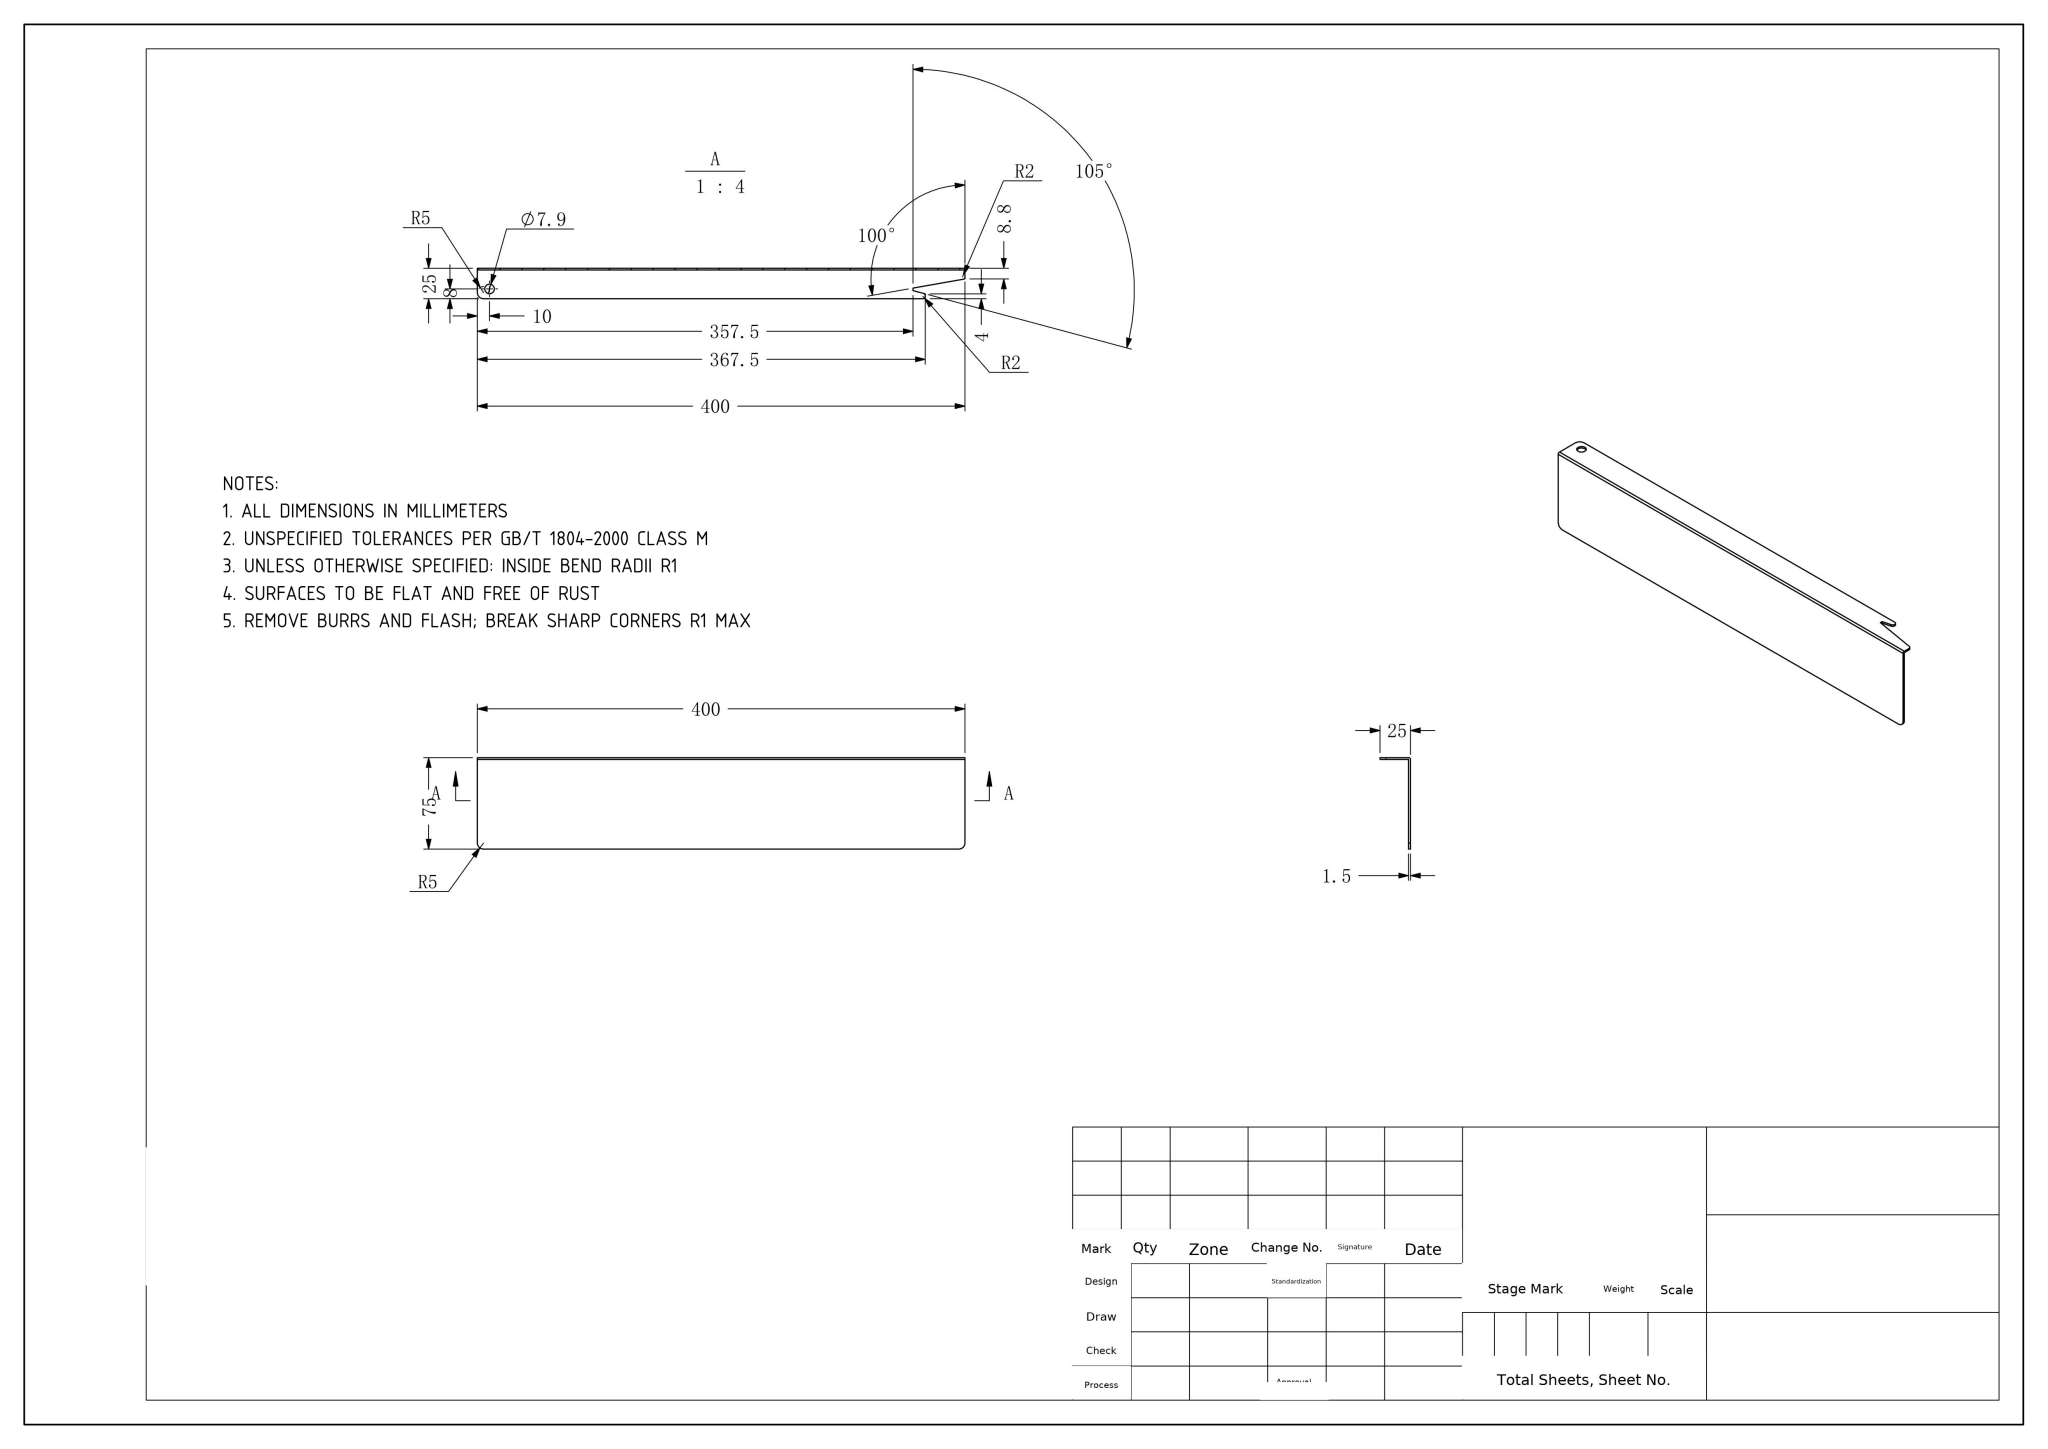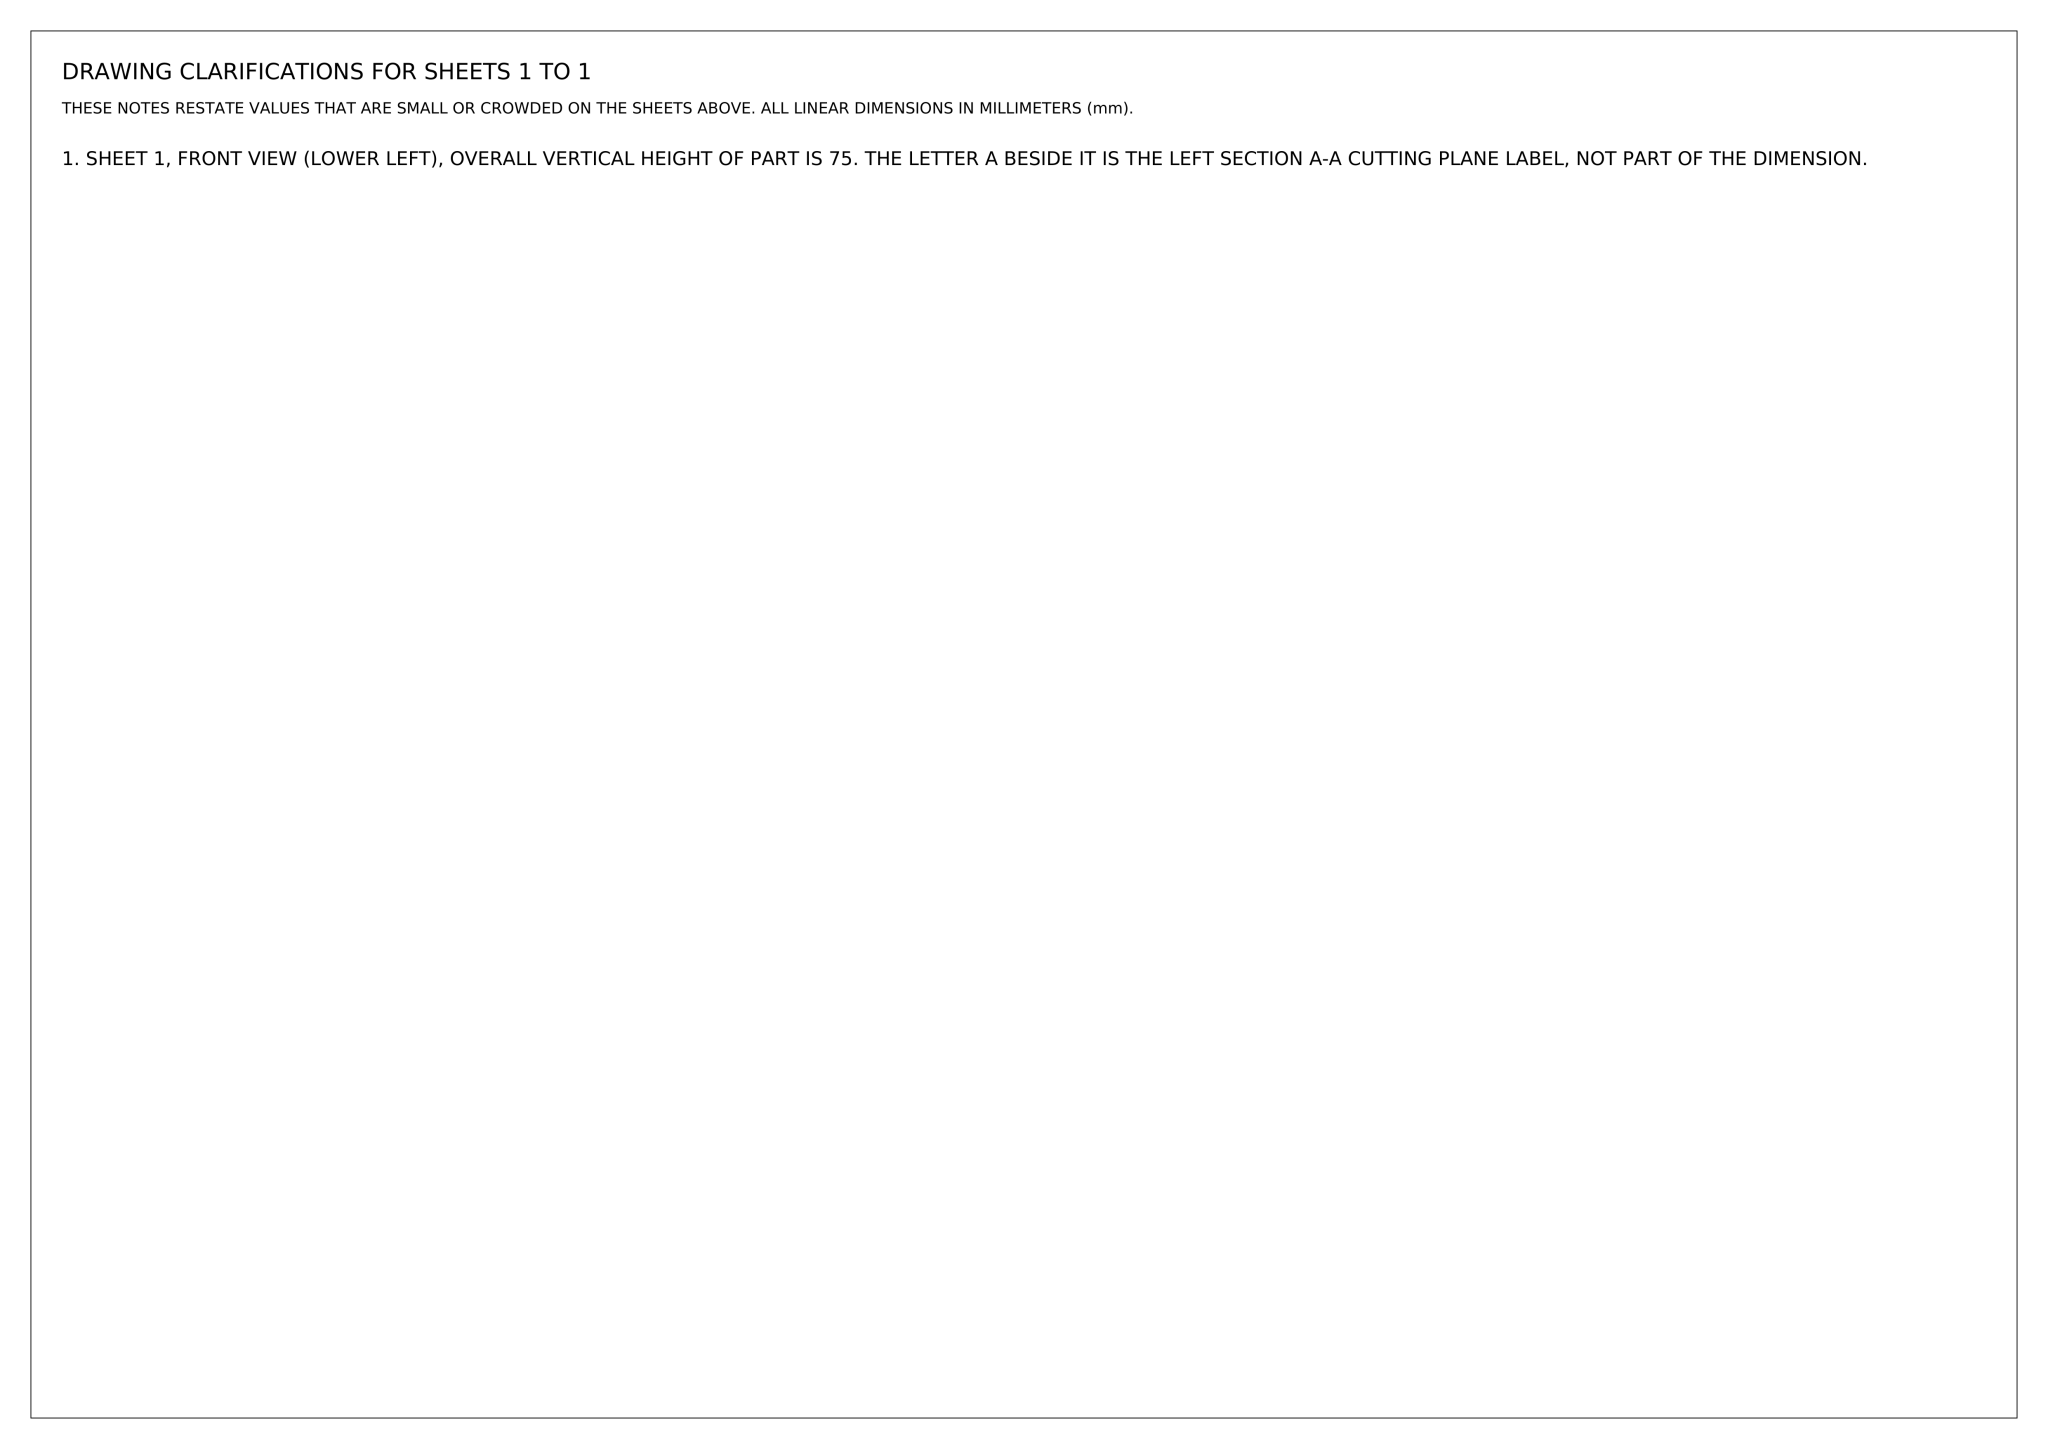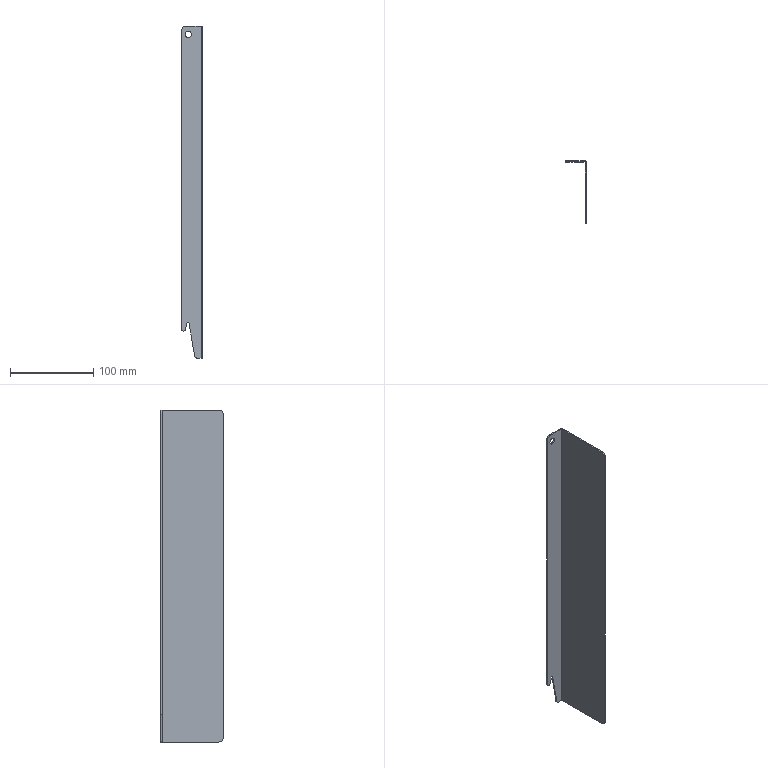Part | NX | mm | Angled Metal Baffle Bracket | 1 solid | 22 faces | box 25 x 75 x 400 mm | volume 58093 mm3 | plane 12 | cylinder 10 | commonest cylinder face diameters 10 x3 4 x3 7.9 x2 3.004 x1 0.004 x1
STEP:
#1=COLOUR_RGB('',0.7529,0.7529,0.7529);
#2=FILL_AREA_STYLE_COLOUR('',#1);
#3=FILL_AREA_STYLE('',(#2));
#4=SURFACE_STYLE_FILL_AREA(#3);
#5=SURFACE_SIDE_STYLE('',(#4));
#6=SURFACE_STYLE_USAGE(.BOTH.,#5);
#7=PRESENTATION_STYLE_ASSIGNMENT((#6));
#8=CARTESIAN_POINT('',(-33.5,-17.5,-31.95));
#9=VERTEX_POINT('',#8);
#10=CARTESIAN_POINT('',(-33.5,-17.5,-24.05));
#11=VERTEX_POINT('',#10);
#12=CARTESIAN_POINT('',(-33.5,-17.5,-28.));
#13=DIRECTION('',(0.,1.,0.));
#14=DIRECTION('',(0.,0.,-1.));
#15=AXIS2_PLACEMENT_3D('',#12,#13,#14);
#16=CIRCLE('',#15,3.95);
#17=EDGE_CURVE('',#9,#11,#16,.T.);
#18=ORIENTED_EDGE('',*,*,#17,.T.);
#19=CARTESIAN_POINT('',(-33.5,-19.,-24.05));
#20=VERTEX_POINT('',#19);
#21=CARTESIAN_POINT('',(-33.5,-17.5,-24.05));
#22=DIRECTION('',(0.,-1.,0.));
#23=VECTOR('',#22,1000.);
#24=LINE('',#21,#23);
#25=EDGE_CURVE('',#11,#20,#24,.T.);
#26=ORIENTED_EDGE('',*,*,#25,.T.);
#27=CARTESIAN_POINT('',(-33.5,-19.,-31.95));
#28=VERTEX_POINT('',#27);
#29=CARTESIAN_POINT('',(-33.5,-19.,-28.));
#30=DIRECTION('',(0.,1.,0.));
#31=DIRECTION('',(0.,0.,-1.));
#32=AXIS2_PLACEMENT_3D('',#29,#30,#31);
#33=CIRCLE('',#32,3.95);
#34=EDGE_CURVE('',#28,#20,#33,.T.);
#35=ORIENTED_EDGE('',*,*,#34,.F.);
#36=CARTESIAN_POINT('',(-33.5,-17.5,-31.95));
#37=DIRECTION('',(0.,-1.,0.));
#38=VECTOR('',#37,1000.);
#39=LINE('',#36,#38);
#40=EDGE_CURVE('',#9,#28,#39,.T.);
#41=ORIENTED_EDGE('',*,*,#40,.F.);
#42=EDGE_LOOP('',(#18,#26,#35,#41));
#43=FACE_OUTER_BOUND('',#42,.T.);
#44=CARTESIAN_POINT('',(-33.5,-17.5,-28.));
#45=DIRECTION('',(0.,-1.,0.));
#46=DIRECTION('',(0.,0.,-1.));
#47=AXIS2_PLACEMENT_3D('',#44,#45,#46);
#48=CYLINDRICAL_SURFACE('',#47,3.95);
#49=ADVANCED_FACE('',(#43),#48,.F.);
#50=CARTESIAN_POINT('',(-18.002,-17.5,-18.));
#51=VERTEX_POINT('',#50);
#52=CARTESIAN_POINT('',(-36.5,-17.5,-18.));
#53=VERTEX_POINT('',#52);
#54=CARTESIAN_POINT('',(-16.5,-17.5,-18.));
#55=DIRECTION('',(-1.,0.,0.));
#56=VECTOR('',#55,1000.);
#57=LINE('',#54,#56);
#58=EDGE_CURVE('',#51,#53,#57,.T.);
#59=ORIENTED_EDGE('',*,*,#58,.T.);
#60=CARTESIAN_POINT('',(-36.5,-19.,-18.));
#61=VERTEX_POINT('',#60);
#62=CARTESIAN_POINT('',(-36.5,-17.5,-18.));
#63=DIRECTION('',(0.,-1.,0.));
#64=VECTOR('',#63,1000.);
#65=LINE('',#62,#64);
#66=EDGE_CURVE('',#53,#61,#65,.T.);
#67=ORIENTED_EDGE('',*,*,#66,.T.);
#68=CARTESIAN_POINT('',(-18.002,-19.,-18.));
#69=VERTEX_POINT('',#68);
#70=CARTESIAN_POINT('',(-16.5,-19.,-18.));
#71=DIRECTION('',(-1.,0.,0.));
#72=VECTOR('',#71,1000.);
#73=LINE('',#70,#72);
#74=EDGE_CURVE('',#69,#61,#73,.T.);
#75=ORIENTED_EDGE('',*,*,#74,.F.);
#76=CARTESIAN_POINT('',(-18.,-19.002,-18.));
#77=VERTEX_POINT('',#76);
#78=CARTESIAN_POINT('',(-18.002,-19.002,-18.));
#79=DIRECTION('',(0.,0.,1.));
#80=DIRECTION('',(-1.,0.,0.));
#81=AXIS2_PLACEMENT_3D('',#78,#79,#80);
#82=CIRCLE('',#81,0.002);
#83=EDGE_CURVE('',#77,#69,#82,.T.);
#84=ORIENTED_EDGE('',*,*,#83,.F.);
#85=CARTESIAN_POINT('',(-18.,-87.5,-18.));
#86=VERTEX_POINT('',#85);
#87=CARTESIAN_POINT('',(-18.,-17.5,-18.));
#88=DIRECTION('',(-0.,1.,0.));
#89=VECTOR('',#88,1000.);
#90=LINE('',#87,#89);
#91=EDGE_CURVE('',#86,#77,#90,.T.);
#92=ORIENTED_EDGE('',*,*,#91,.F.);
#93=CARTESIAN_POINT('',(-16.5,-87.5,-18.));
#94=VERTEX_POINT('',#93);
#95=CARTESIAN_POINT('',(-16.5,-87.5,-18.));
#96=DIRECTION('',(1.,0.,0.));
#97=VECTOR('',#96,1000.);
#98=LINE('',#95,#97);
#99=EDGE_CURVE('',#86,#94,#98,.T.);
#100=ORIENTED_EDGE('',*,*,#99,.T.);
#101=CARTESIAN_POINT('',(-16.5,-19.002,-18.));
#102=VERTEX_POINT('',#101);
#103=CARTESIAN_POINT('',(-16.5,-17.5,-18.));
#104=DIRECTION('',(-0.,1.,0.));
#105=VECTOR('',#104,1000.);
#106=LINE('',#103,#105);
#107=EDGE_CURVE('',#94,#102,#106,.T.);
#108=ORIENTED_EDGE('',*,*,#107,.T.);
#109=CARTESIAN_POINT('',(-18.002,-19.002,-18.));
#110=DIRECTION('',(0.,0.,1.));
#111=DIRECTION('',(-1.,0.,0.));
#112=AXIS2_PLACEMENT_3D('',#109,#110,#111);
#113=CIRCLE('',#112,1.502);
#114=EDGE_CURVE('',#102,#51,#113,.T.);
#115=ORIENTED_EDGE('',*,*,#114,.T.);
#116=EDGE_LOOP('',(#59,#67,#75,#84,#92,#100,#108,#115));
#117=FACE_OUTER_BOUND('',#116,.T.);
#118=CARTESIAN_POINT('',(-16.5,-17.5,-18.));
#119=DIRECTION('',(0.,0.,1.));
#120=DIRECTION('',(-0.,1.,0.));
#121=AXIS2_PLACEMENT_3D('',#118,#119,#120);
#122=PLANE('',#121);
#123=ADVANCED_FACE('',(#117),#122,.T.);
#124=CARTESIAN_POINT('',(-18.,-92.5,-23.));
#125=VERTEX_POINT('',#124);
#126=CARTESIAN_POINT('',(-18.,-92.5,-413.));
#127=VERTEX_POINT('',#126);
#128=CARTESIAN_POINT('',(-18.,-92.5,-18.));
#129=DIRECTION('',(0.,0.,-1.));
#130=VECTOR('',#129,1000.);
#131=LINE('',#128,#130);
#132=EDGE_CURVE('',#125,#127,#131,.T.);
#133=ORIENTED_EDGE('',*,*,#132,.T.);
#134=CARTESIAN_POINT('',(-16.5,-92.5,-413.));
#135=VERTEX_POINT('',#134);
#136=CARTESIAN_POINT('',(-16.5,-92.5,-413.));
#137=DIRECTION('',(1.,0.,0.));
#138=VECTOR('',#137,1000.);
#139=LINE('',#136,#138);
#140=EDGE_CURVE('',#127,#135,#139,.T.);
#141=ORIENTED_EDGE('',*,*,#140,.T.);
#142=CARTESIAN_POINT('',(-16.5,-92.5,-23.));
#143=VERTEX_POINT('',#142);
#144=CARTESIAN_POINT('',(-16.5,-92.5,-18.));
#145=DIRECTION('',(0.,0.,-1.));
#146=VECTOR('',#145,1000.);
#147=LINE('',#144,#146);
#148=EDGE_CURVE('',#143,#135,#147,.T.);
#149=ORIENTED_EDGE('',*,*,#148,.F.);
#150=CARTESIAN_POINT('',(-16.5,-92.5,-23.));
#151=DIRECTION('',(-1.,-0.,0.));
#152=VECTOR('',#151,1000.);
#153=LINE('',#150,#152);
#154=EDGE_CURVE('',#143,#125,#153,.T.);
#155=ORIENTED_EDGE('',*,*,#154,.T.);
#156=EDGE_LOOP('',(#133,#141,#149,#155));
#157=FACE_OUTER_BOUND('',#156,.T.);
#158=CARTESIAN_POINT('',(-16.5,-92.5,-18.));
#159=DIRECTION('',(-0.,1.,0.));
#160=DIRECTION('',(0.,0.,-1.));
#161=AXIS2_PLACEMENT_3D('',#158,#159,#160);
#162=PLANE('',#161);
#163=ADVANCED_FACE('',(#157),#162,.F.);
#164=CARTESIAN_POINT('',(-18.002,-19.,-418.));
#165=VERTEX_POINT('',#164);
#166=CARTESIAN_POINT('',(-23.645,-19.,-418.));
#167=VERTEX_POINT('',#166);
#168=CARTESIAN_POINT('',(-16.5,-19.,-418.));
#169=DIRECTION('',(-1.,0.,0.));
#170=VECTOR('',#169,1000.);
#171=LINE('',#168,#170);
#172=EDGE_CURVE('',#165,#167,#171,.T.);
#173=ORIENTED_EDGE('',*,*,#172,.T.);
#174=CARTESIAN_POINT('',(-23.645,-17.5,-418.));
#175=VERTEX_POINT('',#174);
#176=CARTESIAN_POINT('',(-23.645,-17.5,-418.));
#177=DIRECTION('',(0.,1.,0.));
#178=VECTOR('',#177,1000.);
#179=LINE('',#176,#178);
#180=EDGE_CURVE('',#167,#175,#179,.T.);
#181=ORIENTED_EDGE('',*,*,#180,.T.);
#182=CARTESIAN_POINT('',(-18.002,-17.5,-418.));
#183=VERTEX_POINT('',#182);
#184=CARTESIAN_POINT('',(-16.5,-17.5,-418.));
#185=DIRECTION('',(-1.,0.,0.));
#186=VECTOR('',#185,1000.);
#187=LINE('',#184,#186);
#188=EDGE_CURVE('',#183,#175,#187,.T.);
#189=ORIENTED_EDGE('',*,*,#188,.F.);
#190=CARTESIAN_POINT('',(-16.5,-19.002,-418.));
#191=VERTEX_POINT('',#190);
#192=CARTESIAN_POINT('',(-18.002,-19.002,-418.));
#193=DIRECTION('',(0.,0.,1.));
#194=DIRECTION('',(-1.,0.,0.));
#195=AXIS2_PLACEMENT_3D('',#192,#193,#194);
#196=CIRCLE('',#195,1.502);
#197=EDGE_CURVE('',#191,#183,#196,.T.);
#198=ORIENTED_EDGE('',*,*,#197,.F.);
#199=CARTESIAN_POINT('',(-16.5,-87.5,-418.));
#200=VERTEX_POINT('',#199);
#201=CARTESIAN_POINT('',(-16.5,-17.5,-418.));
#202=DIRECTION('',(-0.,1.,0.));
#203=VECTOR('',#202,1000.);
#204=LINE('',#201,#203);
#205=EDGE_CURVE('',#200,#191,#204,.T.);
#206=ORIENTED_EDGE('',*,*,#205,.F.);
#207=CARTESIAN_POINT('',(-18.,-87.5,-418.));
#208=VERTEX_POINT('',#207);
#209=CARTESIAN_POINT('',(-16.5,-87.5,-418.));
#210=DIRECTION('',(-1.,-0.,0.));
#211=VECTOR('',#210,1000.);
#212=LINE('',#209,#211);
#213=EDGE_CURVE('',#200,#208,#212,.T.);
#214=ORIENTED_EDGE('',*,*,#213,.T.);
#215=CARTESIAN_POINT('',(-18.,-19.002,-418.));
#216=VERTEX_POINT('',#215);
#217=CARTESIAN_POINT('',(-18.,-17.5,-418.));
#218=DIRECTION('',(-0.,1.,0.));
#219=VECTOR('',#218,1000.);
#220=LINE('',#217,#219);
#221=EDGE_CURVE('',#208,#216,#220,.T.);
#222=ORIENTED_EDGE('',*,*,#221,.T.);
#223=CARTESIAN_POINT('',(-18.002,-19.002,-418.));
#224=DIRECTION('',(0.,0.,1.));
#225=DIRECTION('',(-1.,0.,0.));
#226=AXIS2_PLACEMENT_3D('',#223,#224,#225);
#227=CIRCLE('',#226,0.002);
#228=EDGE_CURVE('',#216,#165,#227,.T.);
#229=ORIENTED_EDGE('',*,*,#228,.T.);
#230=EDGE_LOOP('',(#173,#181,#189,#198,#206,#214,#222,#229));
#231=FACE_OUTER_BOUND('',#230,.T.);
#232=CARTESIAN_POINT('',(-16.5,-17.5,-418.));
#233=DIRECTION('',(0.,0.,1.));
#234=DIRECTION('',(-1.,0.,0.));
#235=AXIS2_PLACEMENT_3D('',#232,#233,#234);
#236=PLANE('',#235);
#237=ADVANCED_FACE('',(#231),#236,.F.);
#238=ORIENTED_EDGE('',*,*,#17,.F.);
#239=CARTESIAN_POINT('',(-33.5,-17.5,-28.));
#240=DIRECTION('',(0.,1.,0.));
#241=DIRECTION('',(0.,0.,-1.));
#242=AXIS2_PLACEMENT_3D('',#239,#240,#241);
#243=CIRCLE('',#242,3.95);
#244=EDGE_CURVE('',#11,#9,#243,.T.);
#245=ORIENTED_EDGE('',*,*,#244,.F.);
#246=EDGE_LOOP('',(#238,#245));
#247=FACE_BOUND('',#246,.T.);
#248=CARTESIAN_POINT('',(-39.5,-17.5,-385.479));
#249=VERTEX_POINT('',#248);
#250=CARTESIAN_POINT('',(-39.035,-17.5,-385.479));
#251=VERTEX_POINT('',#250);
#252=CARTESIAN_POINT('',(-16.5,-17.5,-385.479));
#253=DIRECTION('',(1.,0.,0.));
#254=VECTOR('',#253,1000.);
#255=LINE('',#252,#254);
#256=EDGE_CURVE('',#249,#251,#255,.T.);
#257=ORIENTED_EDGE('',*,*,#256,.F.);
#258=CARTESIAN_POINT('',(-41.5,-17.5,-383.479));
#259=VERTEX_POINT('',#258);
#260=CARTESIAN_POINT('',(-39.5,-17.5,-383.479));
#261=DIRECTION('',(0.,1.,0.));
#262=DIRECTION('',(0.,0.,-1.));
#263=AXIS2_PLACEMENT_3D('',#260,#261,#262);
#264=CIRCLE('',#263,2.);
#265=EDGE_CURVE('',#249,#259,#264,.T.);
#266=ORIENTED_EDGE('',*,*,#265,.T.);
#267=CARTESIAN_POINT('',(-41.5,-17.5,-23.));
#268=VERTEX_POINT('',#267);
#269=CARTESIAN_POINT('',(-41.5,-17.5,-18.));
#270=DIRECTION('',(0.,0.,-1.));
#271=VECTOR('',#270,1000.);
#272=LINE('',#269,#271);
#273=EDGE_CURVE('',#268,#259,#272,.T.);
#274=ORIENTED_EDGE('',*,*,#273,.F.);
#275=CARTESIAN_POINT('',(-36.5,-17.5,-23.));
#276=DIRECTION('',(0.,1.,0.));
#277=DIRECTION('',(0.,0.,-1.));
#278=AXIS2_PLACEMENT_3D('',#275,#276,#277);
#279=CIRCLE('',#278,5.);
#280=EDGE_CURVE('',#268,#53,#279,.T.);
#281=ORIENTED_EDGE('',*,*,#280,.T.);
#282=ORIENTED_EDGE('',*,*,#58,.F.);
#283=CARTESIAN_POINT('',(-18.002,-17.5,-18.));
#284=DIRECTION('',(0.,0.,-1.));
#285=VECTOR('',#284,1000.);
#286=LINE('',#283,#285);
#287=EDGE_CURVE('',#51,#183,#286,.T.);
#288=ORIENTED_EDGE('',*,*,#287,.T.);
#289=ORIENTED_EDGE('',*,*,#188,.T.);
#290=CARTESIAN_POINT('',(-25.614,-17.5,-416.347));
#291=VERTEX_POINT('',#290);
#292=CARTESIAN_POINT('',(-23.645,-17.5,-416.));
#293=DIRECTION('',(0.,1.,0.));
#294=DIRECTION('',(0.,0.,-1.));
#295=AXIS2_PLACEMENT_3D('',#292,#293,#294);
#296=CIRCLE('',#295,2.);
#297=EDGE_CURVE('',#175,#291,#296,.T.);
#298=ORIENTED_EDGE('',*,*,#297,.T.);
#299=CARTESIAN_POINT('',(-32.821,-17.5,-375.479));
#300=VERTEX_POINT('',#299);
#301=CARTESIAN_POINT('',(-93.461,-17.5,-31.57));
#302=DIRECTION('',(0.1736,0.,-0.9848));
#303=VECTOR('',#302,1000.);
#304=LINE('',#301,#303);
#305=EDGE_CURVE('',#300,#291,#304,.T.);
#306=ORIENTED_EDGE('',*,*,#305,.F.);
#307=CARTESIAN_POINT('',(-34.821,-17.5,-375.479));
#308=VERTEX_POINT('',#307);
#309=CARTESIAN_POINT('',(-16.5,-17.5,-375.479));
#310=DIRECTION('',(1.,0.,0.));
#311=VECTOR('',#310,1000.);
#312=LINE('',#309,#311);
#313=EDGE_CURVE('',#308,#300,#312,.T.);
#314=ORIENTED_EDGE('',*,*,#313,.F.);
#315=CARTESIAN_POINT('',(-37.103,-17.5,-383.997));
#316=VERTEX_POINT('',#315);
#317=CARTESIAN_POINT('',(55.776,-17.5,-37.366));
#318=DIRECTION('',(0.2588,0.,0.9659));
#319=VECTOR('',#318,1000.);
#320=LINE('',#317,#319);
#321=EDGE_CURVE('',#316,#308,#320,.T.);
#322=ORIENTED_EDGE('',*,*,#321,.F.);
#323=CARTESIAN_POINT('',(-39.035,-17.5,-383.479));
#324=DIRECTION('',(0.,1.,0.));
#325=DIRECTION('',(-0.,0.,-1.));
#326=AXIS2_PLACEMENT_3D('',#323,#324,#325);
#327=CIRCLE('',#326,2.);
#328=EDGE_CURVE('',#316,#251,#327,.T.);
#329=ORIENTED_EDGE('',*,*,#328,.T.);
#330=EDGE_LOOP('',(#257,#266,#274,#281,#282,#288,#289,#298,#306,#314,#322,#329));
#331=FACE_OUTER_BOUND('',#330,.T.);
#332=CARTESIAN_POINT('',(-16.5,-17.5,-18.));
#333=DIRECTION('',(0.,-1.,0.));
#334=DIRECTION('',(0.,0.,-1.));
#335=AXIS2_PLACEMENT_3D('',#332,#333,#334);
#336=PLANE('',#335);
#337=ADVANCED_FACE('',(#247,#331),#336,.F.);
#338=ORIENTED_EDGE('',*,*,#148,.T.);
#339=CARTESIAN_POINT('',(-16.5,-87.5,-413.));
#340=DIRECTION('',(1.,0.,0.));
#341=DIRECTION('',(0.,-1.,0.));
#342=AXIS2_PLACEMENT_3D('',#339,#340,#341);
#343=CIRCLE('',#342,5.);
#344=EDGE_CURVE('',#135,#200,#343,.T.);
#345=ORIENTED_EDGE('',*,*,#344,.T.);
#346=ORIENTED_EDGE('',*,*,#205,.T.);
#347=CARTESIAN_POINT('',(-16.5,-19.002,-18.));
#348=DIRECTION('',(0.,0.,-1.));
#349=VECTOR('',#348,1000.);
#350=LINE('',#347,#349);
#351=EDGE_CURVE('',#102,#191,#350,.T.);
#352=ORIENTED_EDGE('',*,*,#351,.F.);
#353=ORIENTED_EDGE('',*,*,#107,.F.);
#354=CARTESIAN_POINT('',(-16.5,-87.5,-23.));
#355=DIRECTION('',(1.,0.,0.));
#356=DIRECTION('',(0.,-1.,0.));
#357=AXIS2_PLACEMENT_3D('',#354,#355,#356);
#358=CIRCLE('',#357,5.);
#359=EDGE_CURVE('',#94,#143,#358,.T.);
#360=ORIENTED_EDGE('',*,*,#359,.T.);
#361=EDGE_LOOP('',(#338,#345,#346,#352,#353,#360));
#362=FACE_OUTER_BOUND('',#361,.T.);
#363=CARTESIAN_POINT('',(-16.5,-17.5,-18.));
#364=DIRECTION('',(-1.,-0.,0.));
#365=DIRECTION('',(0.,-1.,0.));
#366=AXIS2_PLACEMENT_3D('',#363,#364,#365);
#367=PLANE('',#366);
#368=ADVANCED_FACE('',(#362),#367,.F.);
#369=ORIENTED_EDGE('',*,*,#197,.T.);
#370=ORIENTED_EDGE('',*,*,#287,.F.);
#371=ORIENTED_EDGE('',*,*,#114,.F.);
#372=ORIENTED_EDGE('',*,*,#351,.T.);
#373=EDGE_LOOP('',(#369,#370,#371,#372));
#374=FACE_OUTER_BOUND('',#373,.T.);
#375=CARTESIAN_POINT('',(-18.002,-19.002,-18.));
#376=DIRECTION('',(0.,0.,-1.));
#377=DIRECTION('',(-1.,0.,0.));
#378=AXIS2_PLACEMENT_3D('',#375,#376,#377);
#379=CYLINDRICAL_SURFACE('',#378,1.502);
#380=ADVANCED_FACE('',(#374),#379,.T.);
#381=ORIENTED_EDGE('',*,*,#273,.T.);
#382=CARTESIAN_POINT('',(-41.5,-19.,-383.479));
#383=VERTEX_POINT('',#382);
#384=CARTESIAN_POINT('',(-41.5,-19.,-383.479));
#385=DIRECTION('',(0.,-1.,0.));
#386=VECTOR('',#385,1000.);
#387=LINE('',#384,#386);
#388=EDGE_CURVE('',#259,#383,#387,.T.);
#389=ORIENTED_EDGE('',*,*,#388,.T.);
#390=CARTESIAN_POINT('',(-41.5,-19.,-23.));
#391=VERTEX_POINT('',#390);
#392=CARTESIAN_POINT('',(-41.5,-19.,-18.));
#393=DIRECTION('',(0.,0.,-1.));
#394=VECTOR('',#393,1000.);
#395=LINE('',#392,#394);
#396=EDGE_CURVE('',#391,#383,#395,.T.);
#397=ORIENTED_EDGE('',*,*,#396,.F.);
#398=CARTESIAN_POINT('',(-41.5,-17.5,-23.));
#399=DIRECTION('',(0.,1.,0.));
#400=VECTOR('',#399,1000.);
#401=LINE('',#398,#400);
#402=EDGE_CURVE('',#391,#268,#401,.T.);
#403=ORIENTED_EDGE('',*,*,#402,.T.);
#404=EDGE_LOOP('',(#381,#389,#397,#403));
#405=FACE_OUTER_BOUND('',#404,.T.);
#406=CARTESIAN_POINT('',(-41.5,-17.5,-18.));
#407=DIRECTION('',(-1.,0.,0.));
#408=DIRECTION('',(0.,0.,-1.));
#409=AXIS2_PLACEMENT_3D('',#406,#407,#408);
#410=PLANE('',#409);
#411=ADVANCED_FACE('',(#405),#410,.T.);
#412=ORIENTED_EDGE('',*,*,#396,.T.);
#413=CARTESIAN_POINT('',(-39.5,-19.,-385.479));
#414=VERTEX_POINT('',#413);
#415=CARTESIAN_POINT('',(-39.5,-19.,-383.479));
#416=DIRECTION('',(0.,-1.,0.));
#417=DIRECTION('',(0.,0.,-1.));
#418=AXIS2_PLACEMENT_3D('',#415,#416,#417);
#419=CIRCLE('',#418,2.);
#420=EDGE_CURVE('',#383,#414,#419,.T.);
#421=ORIENTED_EDGE('',*,*,#420,.T.);
#422=CARTESIAN_POINT('',(-39.035,-19.,-385.479));
#423=VERTEX_POINT('',#422);
#424=CARTESIAN_POINT('',(-16.5,-19.,-385.479));
#425=DIRECTION('',(1.,0.,0.));
#426=VECTOR('',#425,1000.);
#427=LINE('',#424,#426);
#428=EDGE_CURVE('',#414,#423,#427,.T.);
#429=ORIENTED_EDGE('',*,*,#428,.T.);
#430=CARTESIAN_POINT('',(-37.103,-19.,-383.997));
#431=VERTEX_POINT('',#430);
#432=CARTESIAN_POINT('',(-39.035,-19.,-383.479));
#433=DIRECTION('',(0.,-1.,0.));
#434=DIRECTION('',(0.,0.,-1.));
#435=AXIS2_PLACEMENT_3D('',#432,#433,#434);
#436=CIRCLE('',#435,2.);
#437=EDGE_CURVE('',#423,#431,#436,.T.);
#438=ORIENTED_EDGE('',*,*,#437,.T.);
#439=CARTESIAN_POINT('',(-34.821,-19.,-375.479));
#440=VERTEX_POINT('',#439);
#441=CARTESIAN_POINT('',(55.776,-19.,-37.366));
#442=DIRECTION('',(0.2588,0.,0.9659));
#443=VECTOR('',#442,1000.);
#444=LINE('',#441,#443);
#445=EDGE_CURVE('',#431,#440,#444,.T.);
#446=ORIENTED_EDGE('',*,*,#445,.T.);
#447=CARTESIAN_POINT('',(-32.821,-19.,-375.479));
#448=VERTEX_POINT('',#447);
#449=CARTESIAN_POINT('',(-16.5,-19.,-375.479));
#450=DIRECTION('',(1.,0.,0.));
#451=VECTOR('',#450,1000.);
#452=LINE('',#449,#451);
#453=EDGE_CURVE('',#440,#448,#452,.T.);
#454=ORIENTED_EDGE('',*,*,#453,.T.);
#455=CARTESIAN_POINT('',(-25.614,-19.,-416.347));
#456=VERTEX_POINT('',#455);
#457=CARTESIAN_POINT('',(-93.461,-19.,-31.57));
#458=DIRECTION('',(0.1736,0.,-0.9848));
#459=VECTOR('',#458,1000.);
#460=LINE('',#457,#459);
#461=EDGE_CURVE('',#448,#456,#460,.T.);
#462=ORIENTED_EDGE('',*,*,#461,.T.);
#463=CARTESIAN_POINT('',(-23.645,-19.,-416.));
#464=DIRECTION('',(0.,-1.,0.));
#465=DIRECTION('',(0.,0.,-1.));
#466=AXIS2_PLACEMENT_3D('',#463,#464,#465);
#467=CIRCLE('',#466,2.);
#468=EDGE_CURVE('',#456,#167,#467,.T.);
#469=ORIENTED_EDGE('',*,*,#468,.T.);
#470=ORIENTED_EDGE('',*,*,#172,.F.);
#471=CARTESIAN_POINT('',(-18.002,-19.,-18.));
#472=DIRECTION('',(0.,0.,-1.));
#473=VECTOR('',#472,1000.);
#474=LINE('',#471,#473);
#475=EDGE_CURVE('',#69,#165,#474,.T.);
#476=ORIENTED_EDGE('',*,*,#475,.F.);
#477=ORIENTED_EDGE('',*,*,#74,.T.);
#478=CARTESIAN_POINT('',(-36.5,-19.,-23.));
#479=DIRECTION('',(0.,-1.,0.));
#480=DIRECTION('',(0.,0.,-1.));
#481=AXIS2_PLACEMENT_3D('',#478,#479,#480);
#482=CIRCLE('',#481,5.);
#483=EDGE_CURVE('',#61,#391,#482,.T.);
#484=ORIENTED_EDGE('',*,*,#483,.T.);
#485=EDGE_LOOP('',(#412,#421,#429,#438,#446,#454,#462,#469,#470,#476,#477,#484));
#486=FACE_OUTER_BOUND('',#485,.T.);
#487=ORIENTED_EDGE('',*,*,#34,.T.);
#488=CARTESIAN_POINT('',(-33.5,-19.,-28.));
#489=DIRECTION('',(0.,1.,0.));
#490=DIRECTION('',(0.,0.,-1.));
#491=AXIS2_PLACEMENT_3D('',#488,#489,#490);
#492=CIRCLE('',#491,3.95);
#493=EDGE_CURVE('',#20,#28,#492,.T.);
#494=ORIENTED_EDGE('',*,*,#493,.T.);
#495=EDGE_LOOP('',(#487,#494));
#496=FACE_BOUND('',#495,.T.);
#497=CARTESIAN_POINT('',(-16.5,-19.,-18.));
#498=DIRECTION('',(0.,-1.,0.));
#499=DIRECTION('',(0.,0.,-1.));
#500=AXIS2_PLACEMENT_3D('',#497,#498,#499);
#501=PLANE('',#500);
#502=ADVANCED_FACE('',(#486,#496),#501,.T.);
#503=ORIENTED_EDGE('',*,*,#221,.F.);
#504=CARTESIAN_POINT('',(-18.,-87.5,-413.));
#505=DIRECTION('',(-1.,-0.,0.));
#506=DIRECTION('',(0.,-1.,0.));
#507=AXIS2_PLACEMENT_3D('',#504,#505,#506);
#508=CIRCLE('',#507,5.);
#509=EDGE_CURVE('',#208,#127,#508,.T.);
#510=ORIENTED_EDGE('',*,*,#509,.T.);
#511=ORIENTED_EDGE('',*,*,#132,.F.);
#512=CARTESIAN_POINT('',(-18.,-87.5,-23.));
#513=DIRECTION('',(-1.,-0.,0.));
#514=DIRECTION('',(0.,-1.,0.));
#515=AXIS2_PLACEMENT_3D('',#512,#513,#514);
#516=CIRCLE('',#515,5.);
#517=EDGE_CURVE('',#125,#86,#516,.T.);
#518=ORIENTED_EDGE('',*,*,#517,.T.);
#519=ORIENTED_EDGE('',*,*,#91,.T.);
#520=CARTESIAN_POINT('',(-18.,-19.002,-18.));
#521=DIRECTION('',(0.,0.,-1.));
#522=VECTOR('',#521,1000.);
#523=LINE('',#520,#522);
#524=EDGE_CURVE('',#77,#216,#523,.T.);
#525=ORIENTED_EDGE('',*,*,#524,.T.);
#526=EDGE_LOOP('',(#503,#510,#511,#518,#519,#525));
#527=FACE_OUTER_BOUND('',#526,.T.);
#528=CARTESIAN_POINT('',(-18.,-17.5,-18.));
#529=DIRECTION('',(-1.,-0.,0.));
#530=DIRECTION('',(0.,-1.,0.));
#531=AXIS2_PLACEMENT_3D('',#528,#529,#530);
#532=PLANE('',#531);
#533=ADVANCED_FACE('',(#527),#532,.T.);
#534=ORIENTED_EDGE('',*,*,#228,.F.);
#535=ORIENTED_EDGE('',*,*,#524,.F.);
#536=ORIENTED_EDGE('',*,*,#83,.T.);
#537=ORIENTED_EDGE('',*,*,#475,.T.);
#538=EDGE_LOOP('',(#534,#535,#536,#537));
#539=FACE_OUTER_BOUND('',#538,.T.);
#540=CARTESIAN_POINT('',(-18.002,-19.002,-18.));
#541=DIRECTION('',(0.,0.,-1.));
#542=DIRECTION('',(-1.,0.,0.));
#543=AXIS2_PLACEMENT_3D('',#540,#541,#542);
#544=CYLINDRICAL_SURFACE('',#543,0.002);
#545=ADVANCED_FACE('',(#539),#544,.F.);
#546=ORIENTED_EDGE('',*,*,#25,.F.);
#547=ORIENTED_EDGE('',*,*,#244,.T.);
#548=ORIENTED_EDGE('',*,*,#40,.T.);
#549=ORIENTED_EDGE('',*,*,#493,.F.);
#550=EDGE_LOOP('',(#546,#547,#548,#549));
#551=FACE_OUTER_BOUND('',#550,.T.);
#552=CARTESIAN_POINT('',(-33.5,-17.5,-28.));
#553=DIRECTION('',(0.,-1.,0.));
#554=DIRECTION('',(0.,0.,-1.));
#555=AXIS2_PLACEMENT_3D('',#552,#553,#554);
#556=CYLINDRICAL_SURFACE('',#555,3.95);
#557=ADVANCED_FACE('',(#551),#556,.F.);
#558=ORIENTED_EDGE('',*,*,#428,.F.);
#559=CARTESIAN_POINT('',(-39.5,-17.5,-385.479));
#560=DIRECTION('',(0.,1.,0.));
#561=VECTOR('',#560,1000.);
#562=LINE('',#559,#561);
#563=EDGE_CURVE('',#414,#249,#562,.T.);
#564=ORIENTED_EDGE('',*,*,#563,.T.);
#565=ORIENTED_EDGE('',*,*,#256,.T.);
#566=CARTESIAN_POINT('',(-39.035,-17.5,-385.479));
#567=DIRECTION('',(0.,-1.,0.));
#568=VECTOR('',#567,1000.);
#569=LINE('',#566,#568);
#570=EDGE_CURVE('',#251,#423,#569,.T.);
#571=ORIENTED_EDGE('',*,*,#570,.T.);
#572=EDGE_LOOP('',(#558,#564,#565,#571));
#573=FACE_OUTER_BOUND('',#572,.T.);
#574=CARTESIAN_POINT('',(-16.5,-17.5,-385.479));
#575=DIRECTION('',(0.,0.,-1.));
#576=DIRECTION('',(1.,0.,0.));
#577=AXIS2_PLACEMENT_3D('',#574,#575,#576);
#578=PLANE('',#577);
#579=ADVANCED_FACE('',(#573),#578,.T.);
#580=ORIENTED_EDGE('',*,*,#445,.F.);
#581=CARTESIAN_POINT('',(-37.103,-17.5,-383.997));
#582=DIRECTION('',(0.,1.,0.));
#583=VECTOR('',#582,1000.);
#584=LINE('',#581,#583);
#585=EDGE_CURVE('',#431,#316,#584,.T.);
#586=ORIENTED_EDGE('',*,*,#585,.T.);
#587=ORIENTED_EDGE('',*,*,#321,.T.);
#588=CARTESIAN_POINT('',(-34.821,-17.5,-375.479));
#589=DIRECTION('',(0.,1.,0.));
#590=VECTOR('',#589,1000.);
#591=LINE('',#588,#590);
#592=EDGE_CURVE('',#440,#308,#591,.T.);
#593=ORIENTED_EDGE('',*,*,#592,.F.);
#594=EDGE_LOOP('',(#580,#586,#587,#593));
#595=FACE_OUTER_BOUND('',#594,.T.);
#596=CARTESIAN_POINT('',(55.776,-17.5,-37.366));
#597=DIRECTION('',(0.9659,0.,-0.2588));
#598=DIRECTION('',(0.2588,0.,0.9659));
#599=AXIS2_PLACEMENT_3D('',#596,#597,#598);
#600=PLANE('',#599);
#601=ADVANCED_FACE('',(#595),#600,.T.);
#602=ORIENTED_EDGE('',*,*,#592,.T.);
#603=ORIENTED_EDGE('',*,*,#313,.T.);
#604=CARTESIAN_POINT('',(-32.821,-17.5,-375.479));
#605=DIRECTION('',(0.,1.,0.));
#606=VECTOR('',#605,1000.);
#607=LINE('',#604,#606);
#608=EDGE_CURVE('',#448,#300,#607,.T.);
#609=ORIENTED_EDGE('',*,*,#608,.F.);
#610=ORIENTED_EDGE('',*,*,#453,.F.);
#611=EDGE_LOOP('',(#602,#603,#609,#610));
#612=FACE_OUTER_BOUND('',#611,.T.);
#613=CARTESIAN_POINT('',(-16.5,-17.5,-375.479));
#614=DIRECTION('',(0.,0.,-1.));
#615=DIRECTION('',(1.,0.,0.));
#616=AXIS2_PLACEMENT_3D('',#613,#614,#615);
#617=PLANE('',#616);
#618=ADVANCED_FACE('',(#612),#617,.T.);
#619=ORIENTED_EDGE('',*,*,#305,.T.);
#620=CARTESIAN_POINT('',(-25.614,-19.,-416.347));
#621=DIRECTION('',(0.,-1.,0.));
#622=VECTOR('',#621,1000.);
#623=LINE('',#620,#622);
#624=EDGE_CURVE('',#291,#456,#623,.T.);
#625=ORIENTED_EDGE('',*,*,#624,.T.);
#626=ORIENTED_EDGE('',*,*,#461,.F.);
#627=ORIENTED_EDGE('',*,*,#608,.T.);
#628=EDGE_LOOP('',(#619,#625,#626,#627));
#629=FACE_OUTER_BOUND('',#628,.T.);
#630=CARTESIAN_POINT('',(-93.461,-17.5,-31.57));
#631=DIRECTION('',(-0.9848,0.,-0.1736));
#632=DIRECTION('',(0.1736,0.,-0.9848));
#633=AXIS2_PLACEMENT_3D('',#630,#631,#632);
#634=PLANE('',#633);
#635=ADVANCED_FACE('',(#629),#634,.T.);
#636=ORIENTED_EDGE('',*,*,#509,.F.);
#637=ORIENTED_EDGE('',*,*,#213,.F.);
#638=ORIENTED_EDGE('',*,*,#344,.F.);
#639=ORIENTED_EDGE('',*,*,#140,.F.);
#640=EDGE_LOOP('',(#636,#637,#638,#639));
#641=FACE_OUTER_BOUND('',#640,.T.);
#642=CARTESIAN_POINT('',(-16.5,-87.5,-413.));
#643=DIRECTION('',(1.,0.,0.));
#644=DIRECTION('',(0.,1.,0.));
#645=AXIS2_PLACEMENT_3D('',#642,#643,#644);
#646=CYLINDRICAL_SURFACE('',#645,5.);
#647=ADVANCED_FACE('',(#641),#646,.T.);
#648=ORIENTED_EDGE('',*,*,#483,.F.);
#649=ORIENTED_EDGE('',*,*,#66,.F.);
#650=ORIENTED_EDGE('',*,*,#280,.F.);
#651=ORIENTED_EDGE('',*,*,#402,.F.);
#652=EDGE_LOOP('',(#648,#649,#650,#651));
#653=FACE_OUTER_BOUND('',#652,.T.);
#654=CARTESIAN_POINT('',(-36.5,-17.5,-23.));
#655=DIRECTION('',(0.,1.,0.));
#656=DIRECTION('',(0.,0.,1.));
#657=AXIS2_PLACEMENT_3D('',#654,#655,#656);
#658=CYLINDRICAL_SURFACE('',#657,5.);
#659=ADVANCED_FACE('',(#653),#658,.T.);
#660=ORIENTED_EDGE('',*,*,#517,.F.);
#661=ORIENTED_EDGE('',*,*,#154,.F.);
#662=ORIENTED_EDGE('',*,*,#359,.F.);
#663=ORIENTED_EDGE('',*,*,#99,.F.);
#664=EDGE_LOOP('',(#660,#661,#662,#663));
#665=FACE_OUTER_BOUND('',#664,.T.);
#666=CARTESIAN_POINT('',(-16.5,-87.5,-23.));
#667=DIRECTION('',(-1.,-0.,0.));
#668=DIRECTION('',(0.,-1.,0.));
#669=AXIS2_PLACEMENT_3D('',#666,#667,#668);
#670=CYLINDRICAL_SURFACE('',#669,5.);
#671=ADVANCED_FACE('',(#665),#670,.T.);
#672=ORIENTED_EDGE('',*,*,#420,.F.);
#673=ORIENTED_EDGE('',*,*,#388,.F.);
#674=ORIENTED_EDGE('',*,*,#265,.F.);
#675=ORIENTED_EDGE('',*,*,#563,.F.);
#676=EDGE_LOOP('',(#672,#673,#674,#675));
#677=FACE_OUTER_BOUND('',#676,.T.);
#678=CARTESIAN_POINT('',(-39.5,-17.5,-383.479));
#679=DIRECTION('',(0.,1.,0.));
#680=DIRECTION('',(0.,0.,1.));
#681=AXIS2_PLACEMENT_3D('',#678,#679,#680);
#682=CYLINDRICAL_SURFACE('',#681,2.);
#683=ADVANCED_FACE('',(#677),#682,.T.);
#684=ORIENTED_EDGE('',*,*,#437,.F.);
#685=ORIENTED_EDGE('',*,*,#570,.F.);
#686=ORIENTED_EDGE('',*,*,#328,.F.);
#687=ORIENTED_EDGE('',*,*,#585,.F.);
#688=EDGE_LOOP('',(#684,#685,#686,#687));
#689=FACE_OUTER_BOUND('',#688,.T.);
#690=CARTESIAN_POINT('',(-39.035,-17.5,-383.479));
#691=DIRECTION('',(0.,1.,0.));
#692=DIRECTION('',(0.,0.,1.));
#693=AXIS2_PLACEMENT_3D('',#690,#691,#692);
#694=CYLINDRICAL_SURFACE('',#693,2.);
#695=ADVANCED_FACE('',(#689),#694,.T.);
#696=ORIENTED_EDGE('',*,*,#468,.F.);
#697=ORIENTED_EDGE('',*,*,#624,.F.);
#698=ORIENTED_EDGE('',*,*,#297,.F.);
#699=ORIENTED_EDGE('',*,*,#180,.F.);
#700=EDGE_LOOP('',(#696,#697,#698,#699));
#701=FACE_OUTER_BOUND('',#700,.T.);
#702=CARTESIAN_POINT('',(-23.645,-17.5,-416.));
#703=DIRECTION('',(0.,-1.,0.));
#704=DIRECTION('',(0.,0.,-1.));
#705=AXIS2_PLACEMENT_3D('',#702,#703,#704);
#706=CYLINDRICAL_SURFACE('',#705,2.);
#707=ADVANCED_FACE('',(#701),#706,.T.);
#708=CLOSED_SHELL('',(#49,#123,#163,#237,#337,#368,#380,#411,#502,#533,#545,#557,#579,#601,#618,#635,#647,#659,#671,#683,#695,#707));
#709=MANIFOLD_SOLID_BREP('',#708);
#710=CARTESIAN_POINT('',(0.,0.,0.));
#711=DIRECTION('',(0.,0.,1.));
#712=DIRECTION('',(1.,0.,0.));
#713=AXIS2_PLACEMENT_3D('',#710,#711,#712);
#714=(LENGTH_UNIT()NAMED_UNIT(*)SI_UNIT(.MILLI.,.METRE.));
#715=UNCERTAINTY_MEASURE_WITH_UNIT(LENGTH_MEASURE(0.00001),#714,'','');
#716=(NAMED_UNIT(*)PLANE_ANGLE_UNIT()SI_UNIT($,.RADIAN.));
#717=(NAMED_UNIT(*)SI_UNIT($,.STERADIAN.)SOLID_ANGLE_UNIT());
#718=(GEOMETRIC_REPRESENTATION_CONTEXT(3)GLOBAL_UNCERTAINTY_ASSIGNED_CONTEXT((#715))GLOBAL_UNIT_ASSIGNED_CONTEXT((#714,#716,#717))REPRESENTATION_CONTEXT('',''));
#719=ADVANCED_BREP_SHAPE_REPRESENTATION('',(#709,#713),#718);
#720=STYLED_ITEM('',(#7),#719);
#721=(LENGTH_UNIT()NAMED_UNIT(*)SI_UNIT(.MILLI.,.METRE.));
#722=UNCERTAINTY_MEASURE_WITH_UNIT(LENGTH_MEASURE(0.00001),#721,'','');
#723=(NAMED_UNIT(*)PLANE_ANGLE_UNIT()SI_UNIT($,.RADIAN.));
#724=(NAMED_UNIT(*)SI_UNIT($,.STERADIAN.)SOLID_ANGLE_UNIT());
#725=(GEOMETRIC_REPRESENTATION_CONTEXT(3)GLOBAL_UNCERTAINTY_ASSIGNED_CONTEXT((#722))GLOBAL_UNIT_ASSIGNED_CONTEXT((#721,#723,#724))REPRESENTATION_CONTEXT('',''));
#726=MECHANICAL_DESIGN_GEOMETRIC_PRESENTATION_REPRESENTATION('',(#720),#725);
#727=PRESENTATION_LAYER_ASSIGNMENT('','',(#720));
#728=COLOUR_RGB('',0.7529,0.7529,0.7529);
#729=FILL_AREA_STYLE_COLOUR('',#728);
#730=FILL_AREA_STYLE('',(#729));
#731=SURFACE_STYLE_FILL_AREA(#730);
#732=SURFACE_SIDE_STYLE('',(#731));
#733=SURFACE_STYLE_USAGE(.BOTH.,#732);
#734=PRESENTATION_STYLE_ASSIGNMENT((#733));
#735=STYLED_ITEM('',(#734),#709);
#736=(LENGTH_UNIT()NAMED_UNIT(*)SI_UNIT(.MILLI.,.METRE.));
#737=UNCERTAINTY_MEASURE_WITH_UNIT(LENGTH_MEASURE(0.00001),#736,'','');
#738=(NAMED_UNIT(*)PLANE_ANGLE_UNIT()SI_UNIT($,.RADIAN.));
#739=(NAMED_UNIT(*)SI_UNIT($,.STERADIAN.)SOLID_ANGLE_UNIT());
#740=(GEOMETRIC_REPRESENTATION_CONTEXT(3)GLOBAL_UNCERTAINTY_ASSIGNED_CONTEXT((#737))GLOBAL_UNIT_ASSIGNED_CONTEXT((#736,#738,#739))REPRESENTATION_CONTEXT('',''));
#741=MECHANICAL_DESIGN_GEOMETRIC_PRESENTATION_REPRESENTATION('',(#735),#740);
#742=PRESENTATION_LAYER_ASSIGNMENT('','',(#735));